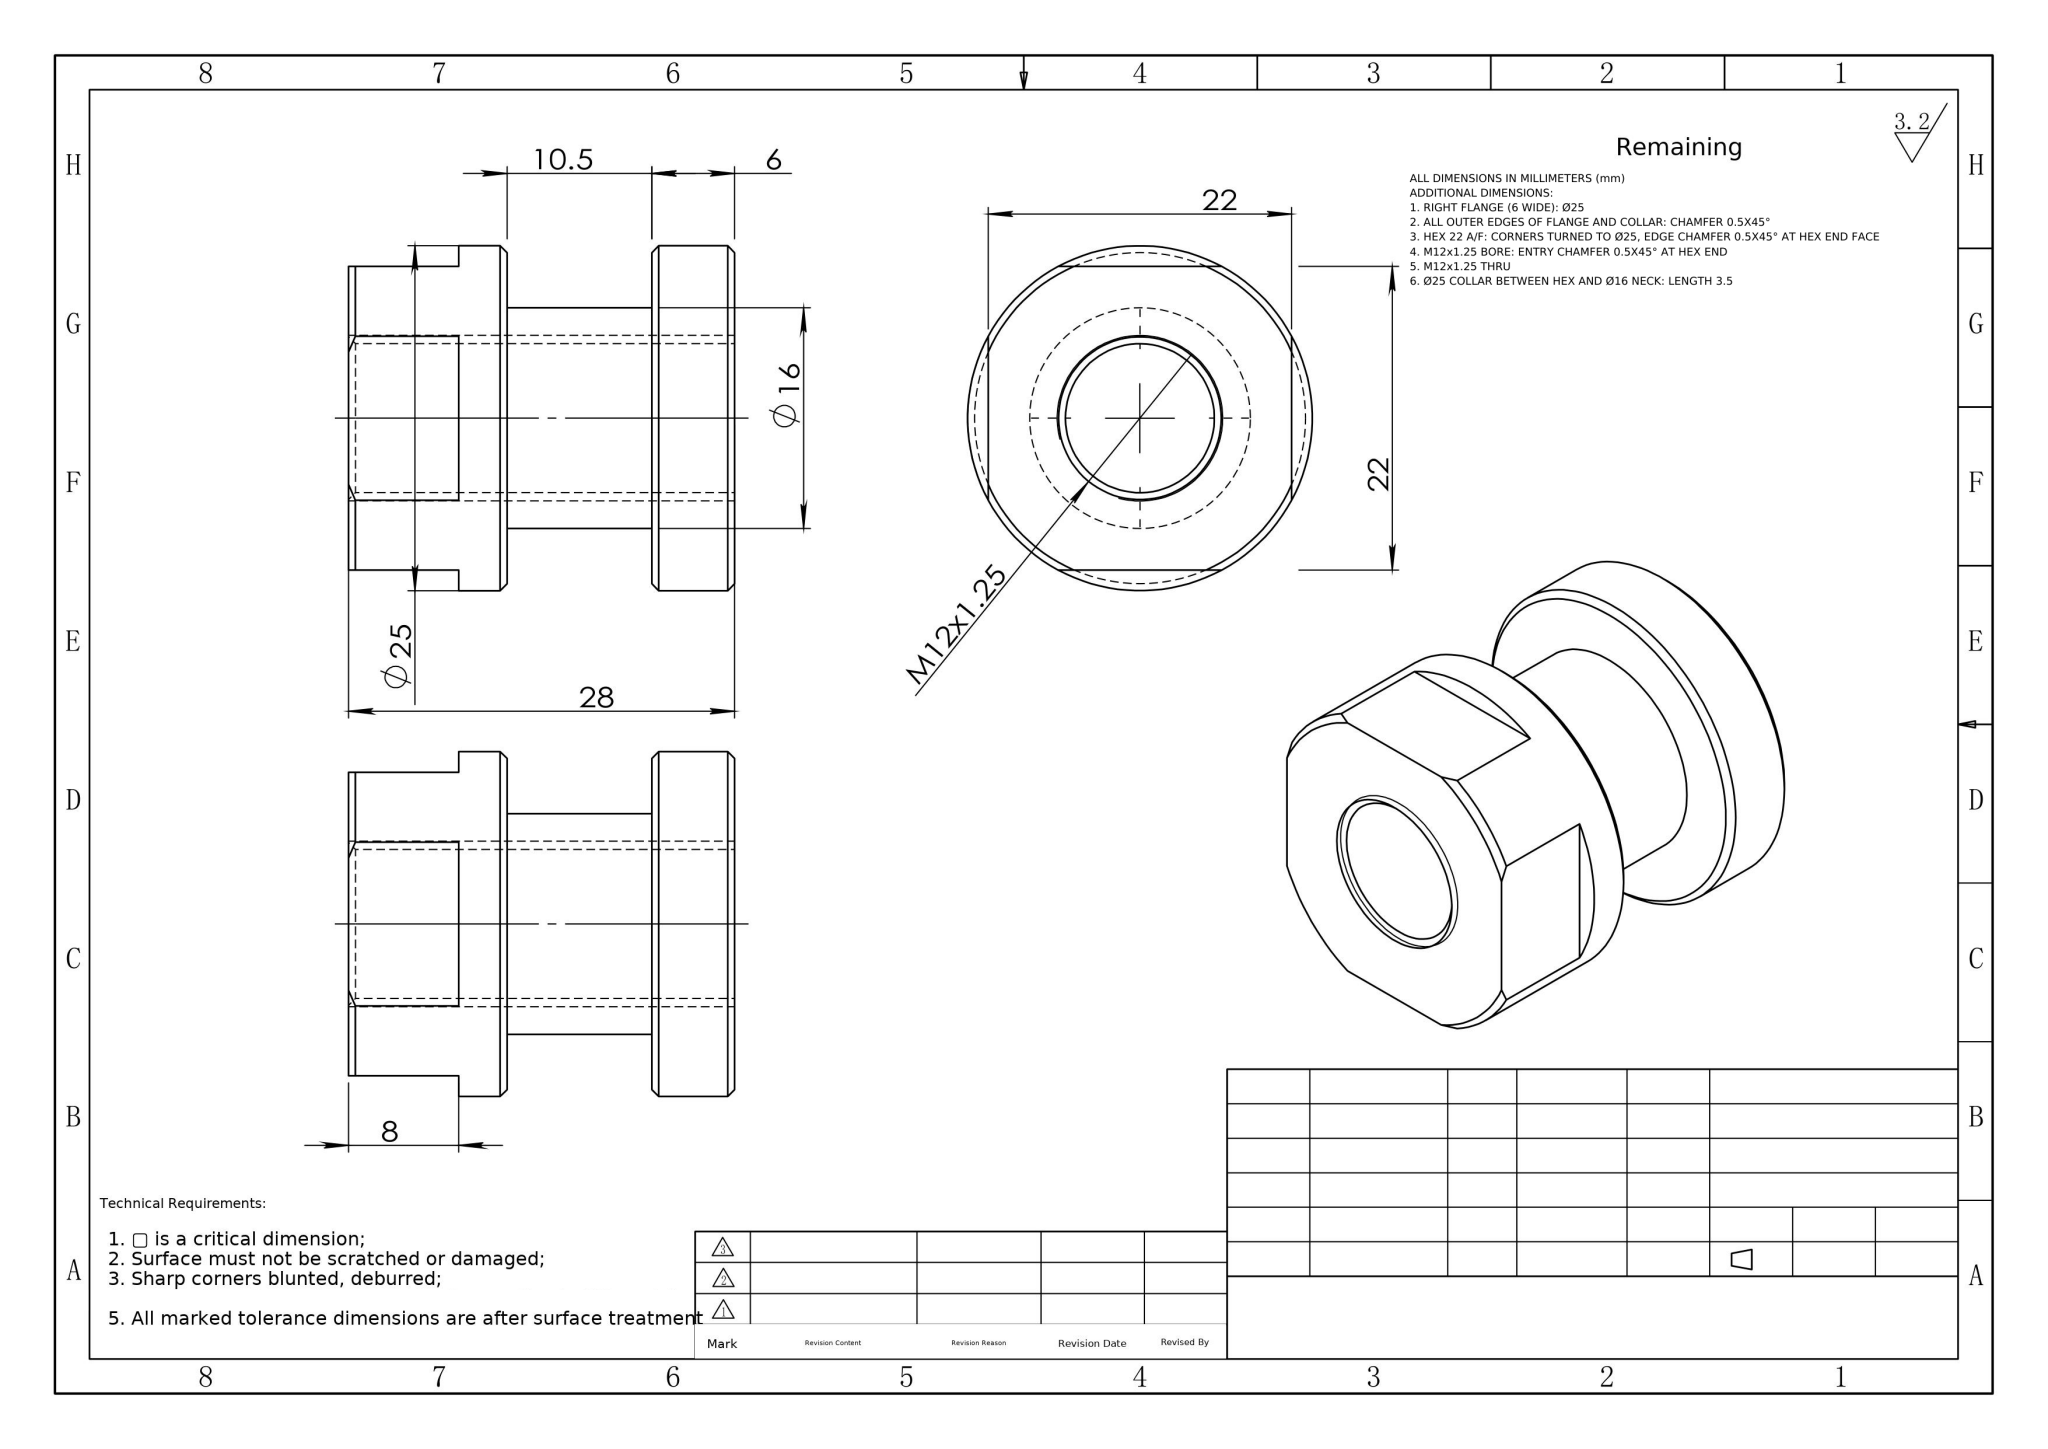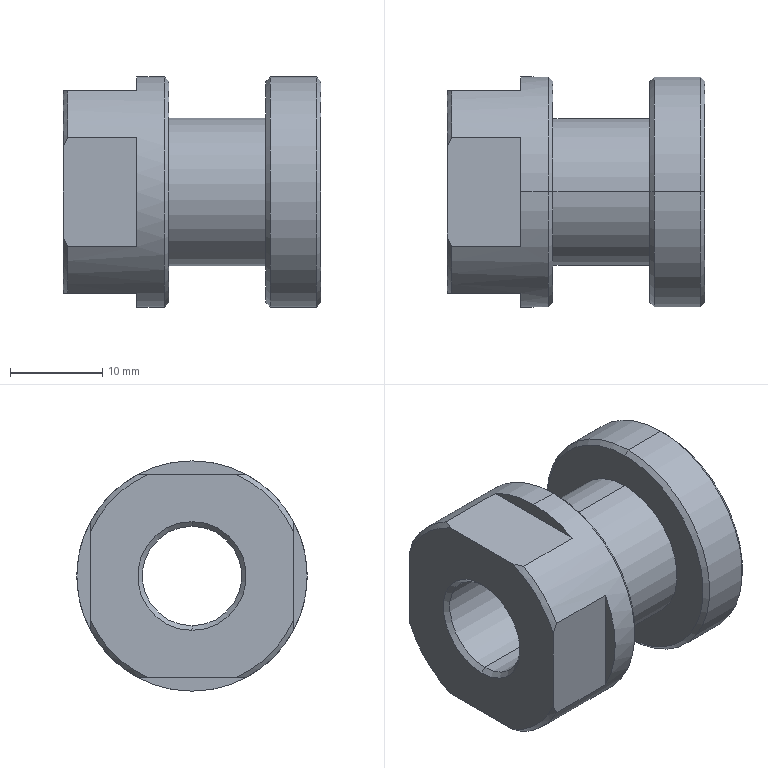Part | NX | mm | 1 solid | 32 faces | box 28 x 25 x 25 mm | volume 7714 mm3 | cone 12 | plane 12 | cylinder 8 | commonest cylinder face diameters 25 x4 10.8 x2 16 x2
STEP:
#1=CARTESIAN_POINT('',(-13.5,0.,-5.4));
#2=VERTEX_POINT('',#1);
#3=CARTESIAN_POINT('',(-13.5,0.,5.4));
#4=VERTEX_POINT('',#3);
#5=CARTESIAN_POINT('',(-13.5,0.,0.));
#6=DIRECTION('',(-1.,0.,0.));
#7=DIRECTION('',(0.,0.,-1.));
#8=AXIS2_PLACEMENT_3D('',#5,#6,#7);
#9=CIRCLE('',#8,5.4);
#10=EDGE_CURVE('',#2,#4,#9,.T.);
#11=ORIENTED_EDGE('',*,*,#10,.F.);
#12=CARTESIAN_POINT('',(-14.,0.,-5.9));
#13=VERTEX_POINT('',#12);
#14=CARTESIAN_POINT('',(-13.5,0.,-5.4));
#15=DIRECTION('',(-0.7071,0.,-0.7071));
#16=VECTOR('',#15,1000.);
#17=LINE('',#14,#16);
#18=EDGE_CURVE('',#2,#13,#17,.T.);
#19=ORIENTED_EDGE('',*,*,#18,.T.);
#20=CARTESIAN_POINT('',(-14.,0.,5.9));
#21=VERTEX_POINT('',#20);
#22=CARTESIAN_POINT('',(-14.,0.,0.));
#23=DIRECTION('',(1.,0.,0.));
#24=DIRECTION('',(0.,0.,-1.));
#25=AXIS2_PLACEMENT_3D('',#22,#23,#24);
#26=CIRCLE('',#25,5.9);
#27=EDGE_CURVE('',#21,#13,#26,.T.);
#28=ORIENTED_EDGE('',*,*,#27,.F.);
#29=CARTESIAN_POINT('',(-13.5,0.,5.4));
#30=DIRECTION('',(-0.7071,0.,0.7071));
#31=VECTOR('',#30,1000.);
#32=LINE('',#29,#31);
#33=EDGE_CURVE('',#4,#21,#32,.T.);
#34=ORIENTED_EDGE('',*,*,#33,.F.);
#35=EDGE_LOOP('',(#11,#19,#28,#34));
#36=FACE_OUTER_BOUND('',#35,.T.);
#37=CARTESIAN_POINT('',(-13.5,0.,0.));
#38=DIRECTION('',(-1.,0.,0.));
#39=DIRECTION('',(0.,0.,1.));
#40=AXIS2_PLACEMENT_3D('',#37,#38,#39);
#41=CONICAL_SURFACE('',#40,5.4,0.7854);
#42=ADVANCED_FACE('',(#36),#41,.F.);
#43=CARTESIAN_POINT('',(8.,0.,12.));
#44=VERTEX_POINT('',#43);
#45=CARTESIAN_POINT('',(8.,0.,-12.));
#46=VERTEX_POINT('',#45);
#47=CARTESIAN_POINT('',(8.,0.,0.));
#48=DIRECTION('',(-1.,0.,0.));
#49=DIRECTION('',(0.,0.,-1.));
#50=AXIS2_PLACEMENT_3D('',#47,#48,#49);
#51=CIRCLE('',#50,12.);
#52=EDGE_CURVE('',#44,#46,#51,.T.);
#53=ORIENTED_EDGE('',*,*,#52,.F.);
#54=CARTESIAN_POINT('',(8.5,0.,12.5));
#55=VERTEX_POINT('',#54);
#56=CARTESIAN_POINT('',(8.,0.,12.));
#57=DIRECTION('',(0.7071,0.,0.7071));
#58=VECTOR('',#57,1000.);
#59=LINE('',#56,#58);
#60=EDGE_CURVE('',#44,#55,#59,.T.);
#61=ORIENTED_EDGE('',*,*,#60,.T.);
#62=CARTESIAN_POINT('',(8.5,0.,-12.5));
#63=VERTEX_POINT('',#62);
#64=CARTESIAN_POINT('',(8.5,0.,0.));
#65=DIRECTION('',(1.,0.,0.));
#66=DIRECTION('',(0.,0.,-1.));
#67=AXIS2_PLACEMENT_3D('',#64,#65,#66);
#68=CIRCLE('',#67,12.5);
#69=EDGE_CURVE('',#63,#55,#68,.T.);
#70=ORIENTED_EDGE('',*,*,#69,.F.);
#71=CARTESIAN_POINT('',(8.,0.,-12.));
#72=DIRECTION('',(0.7071,0.,-0.7071));
#73=VECTOR('',#72,1000.);
#74=LINE('',#71,#73);
#75=EDGE_CURVE('',#46,#63,#74,.T.);
#76=ORIENTED_EDGE('',*,*,#75,.F.);
#77=EDGE_LOOP('',(#53,#61,#70,#76));
#78=FACE_OUTER_BOUND('',#77,.T.);
#79=CARTESIAN_POINT('',(8.,0.,0.));
#80=DIRECTION('',(1.,0.,0.));
#81=DIRECTION('',(0.,0.,-1.));
#82=AXIS2_PLACEMENT_3D('',#79,#80,#81);
#83=CONICAL_SURFACE('',#82,12.,0.7854);
#84=ADVANCED_FACE('',(#78),#83,.T.);
#85=CARTESIAN_POINT('',(-2.5,0.,-12.));
#86=VERTEX_POINT('',#85);
#87=CARTESIAN_POINT('',(-2.5,0.,12.));
#88=VERTEX_POINT('',#87);
#89=CARTESIAN_POINT('',(-2.5,0.,0.));
#90=DIRECTION('',(1.,0.,0.));
#91=DIRECTION('',(0.,0.,1.));
#92=AXIS2_PLACEMENT_3D('',#89,#90,#91);
#93=CIRCLE('',#92,12.);
#94=EDGE_CURVE('',#86,#88,#93,.T.);
#95=ORIENTED_EDGE('',*,*,#94,.F.);
#96=CARTESIAN_POINT('',(-3.,0.,-12.5));
#97=VERTEX_POINT('',#96);
#98=CARTESIAN_POINT('',(-3.,0.,-12.5));
#99=DIRECTION('',(-0.7071,0.,-0.7071));
#100=VECTOR('',#99,1000.);
#101=LINE('',#98,#100);
#102=EDGE_CURVE('',#86,#97,#101,.T.);
#103=ORIENTED_EDGE('',*,*,#102,.T.);
#104=CARTESIAN_POINT('',(-3.,0.,12.5));
#105=VERTEX_POINT('',#104);
#106=CARTESIAN_POINT('',(-3.,0.,0.));
#107=DIRECTION('',(-1.,0.,0.));
#108=DIRECTION('',(0.,0.,1.));
#109=AXIS2_PLACEMENT_3D('',#106,#107,#108);
#110=CIRCLE('',#109,12.5);
#111=EDGE_CURVE('',#105,#97,#110,.T.);
#112=ORIENTED_EDGE('',*,*,#111,.F.);
#113=CARTESIAN_POINT('',(-3.,0.,12.5));
#114=DIRECTION('',(-0.7071,0.,0.7071));
#115=VECTOR('',#114,1000.);
#116=LINE('',#113,#115);
#117=EDGE_CURVE('',#88,#105,#116,.T.);
#118=ORIENTED_EDGE('',*,*,#117,.F.);
#119=EDGE_LOOP('',(#95,#103,#112,#118));
#120=FACE_OUTER_BOUND('',#119,.T.);
#121=CARTESIAN_POINT('',(-3.,0.,0.));
#122=DIRECTION('',(-1.,0.,0.));
#123=DIRECTION('',(0.,0.,1.));
#124=AXIS2_PLACEMENT_3D('',#121,#122,#123);
#125=CONICAL_SURFACE('',#124,12.5,0.7854);
#126=ADVANCED_FACE('',(#120),#125,.T.);
#127=CARTESIAN_POINT('',(14.,0.,-12.));
#128=VERTEX_POINT('',#127);
#129=CARTESIAN_POINT('',(14.,0.,12.));
#130=VERTEX_POINT('',#129);
#131=CARTESIAN_POINT('',(14.,0.,0.));
#132=DIRECTION('',(1.,0.,0.));
#133=DIRECTION('',(0.,0.,1.));
#134=AXIS2_PLACEMENT_3D('',#131,#132,#133);
#135=CIRCLE('',#134,12.);
#136=EDGE_CURVE('',#128,#130,#135,.T.);
#137=ORIENTED_EDGE('',*,*,#136,.F.);
#138=CARTESIAN_POINT('',(13.5,0.,-12.5));
#139=VERTEX_POINT('',#138);
#140=CARTESIAN_POINT('',(13.5,0.,-12.5));
#141=DIRECTION('',(-0.7071,0.,-0.7071));
#142=VECTOR('',#141,1000.);
#143=LINE('',#140,#142);
#144=EDGE_CURVE('',#128,#139,#143,.T.);
#145=ORIENTED_EDGE('',*,*,#144,.T.);
#146=CARTESIAN_POINT('',(13.5,0.,12.5));
#147=VERTEX_POINT('',#146);
#148=CARTESIAN_POINT('',(13.5,0.,0.));
#149=DIRECTION('',(-1.,0.,0.));
#150=DIRECTION('',(0.,0.,1.));
#151=AXIS2_PLACEMENT_3D('',#148,#149,#150);
#152=CIRCLE('',#151,12.5);
#153=EDGE_CURVE('',#147,#139,#152,.T.);
#154=ORIENTED_EDGE('',*,*,#153,.F.);
#155=CARTESIAN_POINT('',(13.5,0.,12.5));
#156=DIRECTION('',(-0.7071,0.,0.7071));
#157=VECTOR('',#156,1000.);
#158=LINE('',#155,#157);
#159=EDGE_CURVE('',#130,#147,#158,.T.);
#160=ORIENTED_EDGE('',*,*,#159,.F.);
#161=EDGE_LOOP('',(#137,#145,#154,#160));
#162=FACE_OUTER_BOUND('',#161,.T.);
#163=CARTESIAN_POINT('',(13.5,0.,0.));
#164=DIRECTION('',(-1.,0.,0.));
#165=DIRECTION('',(0.,0.,1.));
#166=AXIS2_PLACEMENT_3D('',#163,#164,#165);
#167=CONICAL_SURFACE('',#166,12.5,0.7854);
#168=ADVANCED_FACE('',(#162),#167,.T.);
#169=CARTESIAN_POINT('',(14.,0.,-5.4));
#170=VERTEX_POINT('',#169);
#171=CARTESIAN_POINT('',(14.,0.,5.4));
#172=VERTEX_POINT('',#171);
#173=CARTESIAN_POINT('',(14.,0.,0.));
#174=DIRECTION('',(-1.,0.,0.));
#175=DIRECTION('',(0.,0.,1.));
#176=AXIS2_PLACEMENT_3D('',#173,#174,#175);
#177=CIRCLE('',#176,5.4);
#178=EDGE_CURVE('',#170,#172,#177,.T.);
#179=ORIENTED_EDGE('',*,*,#178,.F.);
#180=CARTESIAN_POINT('',(-14.,0.,-5.4));
#181=DIRECTION('',(-1.,0.,0.));
#182=VECTOR('',#181,1000.);
#183=LINE('',#180,#182);
#184=EDGE_CURVE('',#170,#2,#183,.T.);
#185=ORIENTED_EDGE('',*,*,#184,.T.);
#186=ORIENTED_EDGE('',*,*,#10,.T.);
#187=CARTESIAN_POINT('',(-14.,0.,5.4));
#188=DIRECTION('',(-1.,0.,0.));
#189=VECTOR('',#188,1000.);
#190=LINE('',#187,#189);
#191=EDGE_CURVE('',#172,#4,#190,.T.);
#192=ORIENTED_EDGE('',*,*,#191,.F.);
#193=EDGE_LOOP('',(#179,#185,#186,#192));
#194=FACE_OUTER_BOUND('',#193,.T.);
#195=CARTESIAN_POINT('',(-14.,0.,0.));
#196=DIRECTION('',(-1.,0.,0.));
#197=DIRECTION('',(0.,0.,1.));
#198=AXIS2_PLACEMENT_3D('',#195,#196,#197);
#199=CYLINDRICAL_SURFACE('',#198,5.4);
#200=ADVANCED_FACE('',(#194),#199,.F.);
#201=ORIENTED_EDGE('',*,*,#153,.T.);
#202=CARTESIAN_POINT('',(-42.189,0.,-12.5));
#203=DIRECTION('',(-1.,0.,0.));
#204=VECTOR('',#203,1000.);
#205=LINE('',#202,#204);
#206=EDGE_CURVE('',#139,#63,#205,.T.);
#207=ORIENTED_EDGE('',*,*,#206,.T.);
#208=ORIENTED_EDGE('',*,*,#69,.T.);
#209=CARTESIAN_POINT('',(-42.189,0.,12.5));
#210=DIRECTION('',(-1.,0.,0.));
#211=VECTOR('',#210,1000.);
#212=LINE('',#209,#211);
#213=EDGE_CURVE('',#147,#55,#212,.T.);
#214=ORIENTED_EDGE('',*,*,#213,.F.);
#215=EDGE_LOOP('',(#201,#207,#208,#214));
#216=FACE_OUTER_BOUND('',#215,.T.);
#217=CARTESIAN_POINT('',(-42.189,0.,0.));
#218=DIRECTION('',(-1.,0.,0.));
#219=DIRECTION('',(0.,0.,1.));
#220=AXIS2_PLACEMENT_3D('',#217,#218,#219);
#221=CYLINDRICAL_SURFACE('',#220,12.5);
#222=ADVANCED_FACE('',(#216),#221,.T.);
#223=CARTESIAN_POINT('',(8.,0.,8.));
#224=VERTEX_POINT('',#223);
#225=CARTESIAN_POINT('',(8.,0.,-8.));
#226=VERTEX_POINT('',#225);
#227=CARTESIAN_POINT('',(8.,0.,0.));
#228=DIRECTION('',(-1.,0.,0.));
#229=DIRECTION('',(0.,0.,1.));
#230=AXIS2_PLACEMENT_3D('',#227,#228,#229);
#231=CIRCLE('',#230,8.);
#232=EDGE_CURVE('',#224,#226,#231,.T.);
#233=ORIENTED_EDGE('',*,*,#232,.T.);
#234=CARTESIAN_POINT('',(-2.5,0.,-8.));
#235=VERTEX_POINT('',#234);
#236=CARTESIAN_POINT('',(-42.189,0.,-8.));
#237=DIRECTION('',(-1.,0.,0.));
#238=VECTOR('',#237,1000.);
#239=LINE('',#236,#238);
#240=EDGE_CURVE('',#226,#235,#239,.T.);
#241=ORIENTED_EDGE('',*,*,#240,.T.);
#242=CARTESIAN_POINT('',(-2.5,0.,8.));
#243=VERTEX_POINT('',#242);
#244=CARTESIAN_POINT('',(-2.5,0.,0.));
#245=DIRECTION('',(-1.,0.,0.));
#246=DIRECTION('',(0.,0.,1.));
#247=AXIS2_PLACEMENT_3D('',#244,#245,#246);
#248=CIRCLE('',#247,8.);
#249=EDGE_CURVE('',#243,#235,#248,.T.);
#250=ORIENTED_EDGE('',*,*,#249,.F.);
#251=CARTESIAN_POINT('',(-42.189,0.,8.));
#252=DIRECTION('',(-1.,0.,0.));
#253=VECTOR('',#252,1000.);
#254=LINE('',#251,#253);
#255=EDGE_CURVE('',#224,#243,#254,.T.);
#256=ORIENTED_EDGE('',*,*,#255,.F.);
#257=EDGE_LOOP('',(#233,#241,#250,#256));
#258=FACE_OUTER_BOUND('',#257,.T.);
#259=CARTESIAN_POINT('',(-42.189,0.,0.));
#260=DIRECTION('',(-1.,0.,0.));
#261=DIRECTION('',(0.,0.,1.));
#262=AXIS2_PLACEMENT_3D('',#259,#260,#261);
#263=CYLINDRICAL_SURFACE('',#262,8.);
#264=ADVANCED_FACE('',(#258),#263,.T.);
#265=ORIENTED_EDGE('',*,*,#111,.T.);
#266=CARTESIAN_POINT('',(-6.,0.,-12.5));
#267=VERTEX_POINT('',#266);
#268=CARTESIAN_POINT('',(-42.189,0.,-12.5));
#269=DIRECTION('',(-1.,0.,0.));
#270=VECTOR('',#269,1000.);
#271=LINE('',#268,#270);
#272=EDGE_CURVE('',#97,#267,#271,.T.);
#273=ORIENTED_EDGE('',*,*,#272,.T.);
#274=CARTESIAN_POINT('',(-6.,5.937,-11.));
#275=VERTEX_POINT('',#274);
#276=CARTESIAN_POINT('',(-6.,0.,0.));
#277=DIRECTION('',(-1.,0.,0.));
#278=DIRECTION('',(0.,0.,1.));
#279=AXIS2_PLACEMENT_3D('',#276,#277,#278);
#280=CIRCLE('',#279,12.5);
#281=EDGE_CURVE('',#275,#267,#280,.T.);
#282=ORIENTED_EDGE('',*,*,#281,.F.);
#283=CARTESIAN_POINT('',(-13.5,5.937,-11.));
#284=VERTEX_POINT('',#283);
#285=CARTESIAN_POINT('',(-42.189,5.937,-11.));
#286=DIRECTION('',(1.,0.,0.));
#287=VECTOR('',#286,1000.);
#288=LINE('',#285,#287);
#289=EDGE_CURVE('',#284,#275,#288,.T.);
#290=ORIENTED_EDGE('',*,*,#289,.F.);
#291=CARTESIAN_POINT('',(-13.5,11.,-5.937));
#292=VERTEX_POINT('',#291);
#293=CARTESIAN_POINT('',(-13.5,0.,0.));
#294=DIRECTION('',(1.,0.,0.));
#295=DIRECTION('',(0.,0.,-1.));
#296=AXIS2_PLACEMENT_3D('',#293,#294,#295);
#297=CIRCLE('',#296,12.5);
#298=EDGE_CURVE('',#284,#292,#297,.T.);
#299=ORIENTED_EDGE('',*,*,#298,.T.);
#300=CARTESIAN_POINT('',(-6.,11.,-5.937));
#301=VERTEX_POINT('',#300);
#302=CARTESIAN_POINT('',(-42.189,11.,-5.937));
#303=DIRECTION('',(-1.,0.,0.));
#304=VECTOR('',#303,1000.);
#305=LINE('',#302,#304);
#306=EDGE_CURVE('',#301,#292,#305,.T.);
#307=ORIENTED_EDGE('',*,*,#306,.F.);
#308=CARTESIAN_POINT('',(-6.,11.,5.937));
#309=VERTEX_POINT('',#308);
#310=CARTESIAN_POINT('',(-6.,0.,0.));
#311=DIRECTION('',(-1.,0.,0.));
#312=DIRECTION('',(0.,0.,1.));
#313=AXIS2_PLACEMENT_3D('',#310,#311,#312);
#314=CIRCLE('',#313,12.5);
#315=EDGE_CURVE('',#309,#301,#314,.T.);
#316=ORIENTED_EDGE('',*,*,#315,.F.);
#317=CARTESIAN_POINT('',(-13.5,11.,5.937));
#318=VERTEX_POINT('',#317);
#319=CARTESIAN_POINT('',(-42.189,11.,5.937));
#320=DIRECTION('',(1.,0.,0.));
#321=VECTOR('',#320,1000.);
#322=LINE('',#319,#321);
#323=EDGE_CURVE('',#318,#309,#322,.T.);
#324=ORIENTED_EDGE('',*,*,#323,.F.);
#325=CARTESIAN_POINT('',(-13.5,5.937,11.));
#326=VERTEX_POINT('',#325);
#327=CARTESIAN_POINT('',(-13.5,0.,0.));
#328=DIRECTION('',(1.,0.,0.));
#329=DIRECTION('',(0.,0.,-1.));
#330=AXIS2_PLACEMENT_3D('',#327,#328,#329);
#331=CIRCLE('',#330,12.5);
#332=EDGE_CURVE('',#318,#326,#331,.T.);
#333=ORIENTED_EDGE('',*,*,#332,.T.);
#334=CARTESIAN_POINT('',(-6.,5.937,11.));
#335=VERTEX_POINT('',#334);
#336=CARTESIAN_POINT('',(-42.189,5.937,11.));
#337=DIRECTION('',(-1.,0.,0.));
#338=VECTOR('',#337,1000.);
#339=LINE('',#336,#338);
#340=EDGE_CURVE('',#335,#326,#339,.T.);
#341=ORIENTED_EDGE('',*,*,#340,.F.);
#342=CARTESIAN_POINT('',(-6.,0.,12.5));
#343=VERTEX_POINT('',#342);
#344=CARTESIAN_POINT('',(-6.,0.,0.));
#345=DIRECTION('',(-1.,0.,0.));
#346=DIRECTION('',(0.,0.,1.));
#347=AXIS2_PLACEMENT_3D('',#344,#345,#346);
#348=CIRCLE('',#347,12.5);
#349=EDGE_CURVE('',#343,#335,#348,.T.);
#350=ORIENTED_EDGE('',*,*,#349,.F.);
#351=CARTESIAN_POINT('',(-42.189,0.,12.5));
#352=DIRECTION('',(-1.,0.,0.));
#353=VECTOR('',#352,1000.);
#354=LINE('',#351,#353);
#355=EDGE_CURVE('',#105,#343,#354,.T.);
#356=ORIENTED_EDGE('',*,*,#355,.F.);
#357=EDGE_LOOP('',(#265,#273,#282,#290,#299,#307,#316,#324,#333,#341,#350,#356));
#358=FACE_OUTER_BOUND('',#357,.T.);
#359=CARTESIAN_POINT('',(-42.189,0.,0.));
#360=DIRECTION('',(-1.,0.,0.));
#361=DIRECTION('',(0.,0.,1.));
#362=AXIS2_PLACEMENT_3D('',#359,#360,#361);
#363=CYLINDRICAL_SURFACE('',#362,12.5);
#364=ADVANCED_FACE('',(#358),#363,.T.);
#365=ORIENTED_EDGE('',*,*,#27,.T.);
#366=CARTESIAN_POINT('',(-14.,0.,0.));
#367=DIRECTION('',(1.,0.,0.));
#368=DIRECTION('',(0.,0.,-1.));
#369=AXIS2_PLACEMENT_3D('',#366,#367,#368);
#370=CIRCLE('',#369,5.9);
#371=EDGE_CURVE('',#13,#21,#370,.T.);
#372=ORIENTED_EDGE('',*,*,#371,.T.);
#373=EDGE_LOOP('',(#365,#372));
#374=FACE_BOUND('',#373,.T.);
#375=CARTESIAN_POINT('',(-14.,4.796,-11.));
#376=VERTEX_POINT('',#375);
#377=CARTESIAN_POINT('',(-14.,-4.796,-11.));
#378=VERTEX_POINT('',#377);
#379=CARTESIAN_POINT('',(-14.,11.,-11.));
#380=DIRECTION('',(0.,-1.,0.));
#381=VECTOR('',#380,1000.);
#382=LINE('',#379,#381);
#383=EDGE_CURVE('',#376,#378,#382,.T.);
#384=ORIENTED_EDGE('',*,*,#383,.T.);
#385=CARTESIAN_POINT('',(-14.,-11.,-4.796));
#386=VERTEX_POINT('',#385);
#387=CARTESIAN_POINT('',(-14.,0.,0.));
#388=DIRECTION('',(-1.,0.,0.));
#389=DIRECTION('',(0.,0.,-1.));
#390=AXIS2_PLACEMENT_3D('',#387,#388,#389);
#391=CIRCLE('',#390,12.);
#392=EDGE_CURVE('',#378,#386,#391,.T.);
#393=ORIENTED_EDGE('',*,*,#392,.T.);
#394=CARTESIAN_POINT('',(-14.,-11.,4.796));
#395=VERTEX_POINT('',#394);
#396=CARTESIAN_POINT('',(-14.,-11.,-11.));
#397=DIRECTION('',(0.,0.,1.));
#398=VECTOR('',#397,1000.);
#399=LINE('',#396,#398);
#400=EDGE_CURVE('',#386,#395,#399,.T.);
#401=ORIENTED_EDGE('',*,*,#400,.T.);
#402=CARTESIAN_POINT('',(-14.,-4.796,11.));
#403=VERTEX_POINT('',#402);
#404=CARTESIAN_POINT('',(-14.,0.,0.));
#405=DIRECTION('',(-1.,0.,0.));
#406=DIRECTION('',(0.,0.,-1.));
#407=AXIS2_PLACEMENT_3D('',#404,#405,#406);
#408=CIRCLE('',#407,12.);
#409=EDGE_CURVE('',#395,#403,#408,.T.);
#410=ORIENTED_EDGE('',*,*,#409,.T.);
#411=CARTESIAN_POINT('',(-14.,4.796,11.));
#412=VERTEX_POINT('',#411);
#413=CARTESIAN_POINT('',(-14.,11.,11.));
#414=DIRECTION('',(0.,1.,-0.));
#415=VECTOR('',#414,1000.);
#416=LINE('',#413,#415);
#417=EDGE_CURVE('',#403,#412,#416,.T.);
#418=ORIENTED_EDGE('',*,*,#417,.T.);
#419=CARTESIAN_POINT('',(-14.,11.,4.796));
#420=VERTEX_POINT('',#419);
#421=CARTESIAN_POINT('',(-14.,0.,0.));
#422=DIRECTION('',(-1.,0.,0.));
#423=DIRECTION('',(0.,0.,-1.));
#424=AXIS2_PLACEMENT_3D('',#421,#422,#423);
#425=CIRCLE('',#424,12.);
#426=EDGE_CURVE('',#412,#420,#425,.T.);
#427=ORIENTED_EDGE('',*,*,#426,.T.);
#428=CARTESIAN_POINT('',(-14.,11.,-4.796));
#429=VERTEX_POINT('',#428);
#430=CARTESIAN_POINT('',(-14.,11.,-11.));
#431=DIRECTION('',(0.,0.,-1.));
#432=VECTOR('',#431,1000.);
#433=LINE('',#430,#432);
#434=EDGE_CURVE('',#420,#429,#433,.T.);
#435=ORIENTED_EDGE('',*,*,#434,.T.);
#436=CARTESIAN_POINT('',(-14.,0.,0.));
#437=DIRECTION('',(-1.,0.,0.));
#438=DIRECTION('',(0.,0.,-1.));
#439=AXIS2_PLACEMENT_3D('',#436,#437,#438);
#440=CIRCLE('',#439,12.);
#441=EDGE_CURVE('',#429,#376,#440,.T.);
#442=ORIENTED_EDGE('',*,*,#441,.T.);
#443=EDGE_LOOP('',(#384,#393,#401,#410,#418,#427,#435,#442));
#444=FACE_OUTER_BOUND('',#443,.T.);
#445=CARTESIAN_POINT('',(-14.,-0.,0.));
#446=DIRECTION('',(1.,0.,0.));
#447=DIRECTION('',(0.,0.,-1.));
#448=AXIS2_PLACEMENT_3D('',#445,#446,#447);
#449=PLANE('',#448);
#450=ADVANCED_FACE('',(#374,#444),#449,.F.);
#451=ORIENTED_EDGE('',*,*,#272,.F.);
#452=CARTESIAN_POINT('',(-3.,0.,0.));
#453=DIRECTION('',(-1.,0.,0.));
#454=DIRECTION('',(0.,0.,1.));
#455=AXIS2_PLACEMENT_3D('',#452,#453,#454);
#456=CIRCLE('',#455,12.5);
#457=EDGE_CURVE('',#97,#105,#456,.T.);
#458=ORIENTED_EDGE('',*,*,#457,.T.);
#459=ORIENTED_EDGE('',*,*,#355,.T.);
#460=CARTESIAN_POINT('',(-6.,-5.937,11.));
#461=VERTEX_POINT('',#460);
#462=CARTESIAN_POINT('',(-6.,0.,0.));
#463=DIRECTION('',(-1.,0.,0.));
#464=DIRECTION('',(0.,0.,1.));
#465=AXIS2_PLACEMENT_3D('',#462,#463,#464);
#466=CIRCLE('',#465,12.5);
#467=EDGE_CURVE('',#461,#343,#466,.T.);
#468=ORIENTED_EDGE('',*,*,#467,.F.);
#469=CARTESIAN_POINT('',(-13.5,-5.937,11.));
#470=VERTEX_POINT('',#469);
#471=CARTESIAN_POINT('',(-42.189,-5.937,11.));
#472=DIRECTION('',(1.,0.,0.));
#473=VECTOR('',#472,1000.);
#474=LINE('',#471,#473);
#475=EDGE_CURVE('',#470,#461,#474,.T.);
#476=ORIENTED_EDGE('',*,*,#475,.F.);
#477=CARTESIAN_POINT('',(-13.5,-11.,5.937));
#478=VERTEX_POINT('',#477);
#479=CARTESIAN_POINT('',(-13.5,0.,0.));
#480=DIRECTION('',(1.,0.,0.));
#481=DIRECTION('',(0.,0.,-1.));
#482=AXIS2_PLACEMENT_3D('',#479,#480,#481);
#483=CIRCLE('',#482,12.5);
#484=EDGE_CURVE('',#470,#478,#483,.T.);
#485=ORIENTED_EDGE('',*,*,#484,.T.);
#486=CARTESIAN_POINT('',(-6.,-11.,5.937));
#487=VERTEX_POINT('',#486);
#488=CARTESIAN_POINT('',(-42.189,-11.,5.937));
#489=DIRECTION('',(-1.,0.,0.));
#490=VECTOR('',#489,1000.);
#491=LINE('',#488,#490);
#492=EDGE_CURVE('',#487,#478,#491,.T.);
#493=ORIENTED_EDGE('',*,*,#492,.F.);
#494=CARTESIAN_POINT('',(-6.,-11.,-5.937));
#495=VERTEX_POINT('',#494);
#496=CARTESIAN_POINT('',(-6.,0.,0.));
#497=DIRECTION('',(-1.,0.,0.));
#498=DIRECTION('',(0.,0.,1.));
#499=AXIS2_PLACEMENT_3D('',#496,#497,#498);
#500=CIRCLE('',#499,12.5);
#501=EDGE_CURVE('',#495,#487,#500,.T.);
#502=ORIENTED_EDGE('',*,*,#501,.F.);
#503=CARTESIAN_POINT('',(-13.5,-11.,-5.937));
#504=VERTEX_POINT('',#503);
#505=CARTESIAN_POINT('',(-42.189,-11.,-5.937));
#506=DIRECTION('',(1.,0.,0.));
#507=VECTOR('',#506,1000.);
#508=LINE('',#505,#507);
#509=EDGE_CURVE('',#504,#495,#508,.T.);
#510=ORIENTED_EDGE('',*,*,#509,.F.);
#511=CARTESIAN_POINT('',(-13.5,-5.937,-11.));
#512=VERTEX_POINT('',#511);
#513=CARTESIAN_POINT('',(-13.5,0.,0.));
#514=DIRECTION('',(1.,0.,0.));
#515=DIRECTION('',(0.,0.,-1.));
#516=AXIS2_PLACEMENT_3D('',#513,#514,#515);
#517=CIRCLE('',#516,12.5);
#518=EDGE_CURVE('',#504,#512,#517,.T.);
#519=ORIENTED_EDGE('',*,*,#518,.T.);
#520=CARTESIAN_POINT('',(-6.,-5.937,-11.));
#521=VERTEX_POINT('',#520);
#522=CARTESIAN_POINT('',(-42.189,-5.937,-11.));
#523=DIRECTION('',(-1.,0.,0.));
#524=VECTOR('',#523,1000.);
#525=LINE('',#522,#524);
#526=EDGE_CURVE('',#521,#512,#525,.T.);
#527=ORIENTED_EDGE('',*,*,#526,.F.);
#528=CARTESIAN_POINT('',(-6.,0.,0.));
#529=DIRECTION('',(-1.,0.,0.));
#530=DIRECTION('',(0.,0.,1.));
#531=AXIS2_PLACEMENT_3D('',#528,#529,#530);
#532=CIRCLE('',#531,12.5);
#533=EDGE_CURVE('',#267,#521,#532,.T.);
#534=ORIENTED_EDGE('',*,*,#533,.F.);
#535=EDGE_LOOP('',(#451,#458,#459,#468,#476,#485,#493,#502,#510,#519,#527,#534));
#536=FACE_OUTER_BOUND('',#535,.T.);
#537=CARTESIAN_POINT('',(-42.189,0.,0.));
#538=DIRECTION('',(-1.,0.,0.));
#539=DIRECTION('',(0.,0.,1.));
#540=AXIS2_PLACEMENT_3D('',#537,#538,#539);
#541=CYLINDRICAL_SURFACE('',#540,12.5);
#542=ADVANCED_FACE('',(#536),#541,.T.);
#543=CARTESIAN_POINT('',(14.,0.,0.));
#544=DIRECTION('',(1.,0.,0.));
#545=DIRECTION('',(0.,0.,1.));
#546=AXIS2_PLACEMENT_3D('',#543,#544,#545);
#547=CIRCLE('',#546,12.);
#548=EDGE_CURVE('',#130,#128,#547,.T.);
#549=ORIENTED_EDGE('',*,*,#548,.T.);
#550=ORIENTED_EDGE('',*,*,#136,.T.);
#551=EDGE_LOOP('',(#549,#550));
#552=FACE_OUTER_BOUND('',#551,.T.);
#553=CARTESIAN_POINT('',(14.,0.,0.));
#554=DIRECTION('',(-1.,0.,0.));
#555=DIRECTION('',(0.,0.,1.));
#556=AXIS2_PLACEMENT_3D('',#553,#554,#555);
#557=CIRCLE('',#556,5.4);
#558=EDGE_CURVE('',#172,#170,#557,.T.);
#559=ORIENTED_EDGE('',*,*,#558,.T.);
#560=ORIENTED_EDGE('',*,*,#178,.T.);
#561=EDGE_LOOP('',(#559,#560));
#562=FACE_BOUND('',#561,.T.);
#563=CARTESIAN_POINT('',(14.,12.5,0.));
#564=DIRECTION('',(-1.,0.,0.));
#565=DIRECTION('',(0.,0.,1.));
#566=AXIS2_PLACEMENT_3D('',#563,#564,#565);
#567=PLANE('',#566);
#568=ADVANCED_FACE('',(#552,#562),#567,.F.);
#569=CARTESIAN_POINT('',(-2.5,0.,0.));
#570=DIRECTION('',(1.,0.,0.));
#571=DIRECTION('',(0.,0.,1.));
#572=AXIS2_PLACEMENT_3D('',#569,#570,#571);
#573=CIRCLE('',#572,12.);
#574=EDGE_CURVE('',#88,#86,#573,.T.);
#575=ORIENTED_EDGE('',*,*,#574,.T.);
#576=ORIENTED_EDGE('',*,*,#94,.T.);
#577=EDGE_LOOP('',(#575,#576));
#578=FACE_OUTER_BOUND('',#577,.T.);
#579=ORIENTED_EDGE('',*,*,#249,.T.);
#580=CARTESIAN_POINT('',(-2.5,0.,0.));
#581=DIRECTION('',(-1.,0.,0.));
#582=DIRECTION('',(0.,0.,1.));
#583=AXIS2_PLACEMENT_3D('',#580,#581,#582);
#584=CIRCLE('',#583,8.);
#585=EDGE_CURVE('',#235,#243,#584,.T.);
#586=ORIENTED_EDGE('',*,*,#585,.T.);
#587=EDGE_LOOP('',(#579,#586));
#588=FACE_BOUND('',#587,.T.);
#589=CARTESIAN_POINT('',(-2.5,12.5,0.));
#590=DIRECTION('',(-1.,0.,0.));
#591=DIRECTION('',(0.,0.,1.));
#592=AXIS2_PLACEMENT_3D('',#589,#590,#591);
#593=PLANE('',#592);
#594=ADVANCED_FACE('',(#578,#588),#593,.F.);
#595=ORIENTED_EDGE('',*,*,#240,.F.);
#596=CARTESIAN_POINT('',(8.,0.,0.));
#597=DIRECTION('',(-1.,0.,0.));
#598=DIRECTION('',(0.,0.,1.));
#599=AXIS2_PLACEMENT_3D('',#596,#597,#598);
#600=CIRCLE('',#599,8.);
#601=EDGE_CURVE('',#226,#224,#600,.T.);
#602=ORIENTED_EDGE('',*,*,#601,.T.);
#603=ORIENTED_EDGE('',*,*,#255,.T.);
#604=ORIENTED_EDGE('',*,*,#585,.F.);
#605=EDGE_LOOP('',(#595,#602,#603,#604));
#606=FACE_OUTER_BOUND('',#605,.T.);
#607=CARTESIAN_POINT('',(-42.189,0.,0.));
#608=DIRECTION('',(-1.,0.,0.));
#609=DIRECTION('',(0.,0.,1.));
#610=AXIS2_PLACEMENT_3D('',#607,#608,#609);
#611=CYLINDRICAL_SURFACE('',#610,8.);
#612=ADVANCED_FACE('',(#606),#611,.T.);
#613=CARTESIAN_POINT('',(8.,0.,0.));
#614=DIRECTION('',(-1.,0.,0.));
#615=DIRECTION('',(0.,0.,-1.));
#616=AXIS2_PLACEMENT_3D('',#613,#614,#615);
#617=CIRCLE('',#616,12.);
#618=EDGE_CURVE('',#46,#44,#617,.T.);
#619=ORIENTED_EDGE('',*,*,#618,.T.);
#620=ORIENTED_EDGE('',*,*,#52,.T.);
#621=EDGE_LOOP('',(#619,#620));
#622=FACE_OUTER_BOUND('',#621,.T.);
#623=ORIENTED_EDGE('',*,*,#232,.F.);
#624=ORIENTED_EDGE('',*,*,#601,.F.);
#625=EDGE_LOOP('',(#623,#624));
#626=FACE_BOUND('',#625,.T.);
#627=CARTESIAN_POINT('',(8.,12.5,0.));
#628=DIRECTION('',(1.,0.,0.));
#629=DIRECTION('',(0.,0.,-1.));
#630=AXIS2_PLACEMENT_3D('',#627,#628,#629);
#631=PLANE('',#630);
#632=ADVANCED_FACE('',(#622,#626),#631,.F.);
#633=ORIENTED_EDGE('',*,*,#206,.F.);
#634=CARTESIAN_POINT('',(13.5,0.,0.));
#635=DIRECTION('',(-1.,0.,0.));
#636=DIRECTION('',(0.,0.,1.));
#637=AXIS2_PLACEMENT_3D('',#634,#635,#636);
#638=CIRCLE('',#637,12.5);
#639=EDGE_CURVE('',#139,#147,#638,.T.);
#640=ORIENTED_EDGE('',*,*,#639,.T.);
#641=ORIENTED_EDGE('',*,*,#213,.T.);
#642=CARTESIAN_POINT('',(8.5,0.,0.));
#643=DIRECTION('',(1.,0.,0.));
#644=DIRECTION('',(0.,0.,-1.));
#645=AXIS2_PLACEMENT_3D('',#642,#643,#644);
#646=CIRCLE('',#645,12.5);
#647=EDGE_CURVE('',#55,#63,#646,.T.);
#648=ORIENTED_EDGE('',*,*,#647,.T.);
#649=EDGE_LOOP('',(#633,#640,#641,#648));
#650=FACE_OUTER_BOUND('',#649,.T.);
#651=CARTESIAN_POINT('',(-42.189,0.,0.));
#652=DIRECTION('',(-1.,0.,0.));
#653=DIRECTION('',(0.,0.,1.));
#654=AXIS2_PLACEMENT_3D('',#651,#652,#653);
#655=CYLINDRICAL_SURFACE('',#654,12.5);
#656=ADVANCED_FACE('',(#650),#655,.T.);
#657=ORIENTED_EDGE('',*,*,#306,.T.);
#658=CARTESIAN_POINT('',(-13.5,11.,-5.937));
#659=CARTESIAN_POINT('',(-13.678,11.,-5.562));
#660=CARTESIAN_POINT('',(-13.846,11.,-5.182));
#661=CARTESIAN_POINT('',(-14.,11.,-4.796));
#662=B_SPLINE_CURVE_WITH_KNOTS('',3,(#658,#659,#660,#661),.UNSPECIFIED.,.F.,.F.,(4,4),(0.,0.001246),.UNSPECIFIED.);
#663=EDGE_CURVE('',#292,#429,#662,.T.);
#664=ORIENTED_EDGE('',*,*,#663,.T.);
#665=ORIENTED_EDGE('',*,*,#434,.F.);
#666=CARTESIAN_POINT('',(-14.,11.,4.796));
#667=CARTESIAN_POINT('',(-13.846,11.,5.182));
#668=CARTESIAN_POINT('',(-13.678,11.,5.562));
#669=CARTESIAN_POINT('',(-13.5,11.,5.937));
#670=B_SPLINE_CURVE_WITH_KNOTS('',3,(#666,#667,#668,#669),.UNSPECIFIED.,.F.,.F.,(4,4),(0.,0.001246),.UNSPECIFIED.);
#671=EDGE_CURVE('',#420,#318,#670,.T.);
#672=ORIENTED_EDGE('',*,*,#671,.T.);
#673=ORIENTED_EDGE('',*,*,#323,.T.);
#674=CARTESIAN_POINT('',(-6.,11.,-11.));
#675=DIRECTION('',(0.,0.,-1.));
#676=VECTOR('',#675,1000.);
#677=LINE('',#674,#676);
#678=EDGE_CURVE('',#309,#301,#677,.T.);
#679=ORIENTED_EDGE('',*,*,#678,.T.);
#680=EDGE_LOOP('',(#657,#664,#665,#672,#673,#679));
#681=FACE_OUTER_BOUND('',#680,.T.);
#682=CARTESIAN_POINT('',(-6.,11.,-11.));
#683=DIRECTION('',(0.,1.,0.));
#684=DIRECTION('',(0.,0.,1.));
#685=AXIS2_PLACEMENT_3D('',#682,#683,#684);
#686=PLANE('',#685);
#687=ADVANCED_FACE('',(#681),#686,.T.);
#688=ORIENTED_EDGE('',*,*,#315,.T.);
#689=ORIENTED_EDGE('',*,*,#678,.F.);
#690=EDGE_LOOP('',(#688,#689));
#691=FACE_OUTER_BOUND('',#690,.T.);
#692=CARTESIAN_POINT('',(-6.,0.,0.));
#693=DIRECTION('',(-1.,0.,0.));
#694=DIRECTION('',(0.,0.,1.));
#695=AXIS2_PLACEMENT_3D('',#692,#693,#694);
#696=PLANE('',#695);
#697=ADVANCED_FACE('',(#691),#696,.T.);
#698=ORIENTED_EDGE('',*,*,#526,.T.);
#699=CARTESIAN_POINT('',(-13.5,-5.937,-11.));
#700=CARTESIAN_POINT('',(-13.678,-5.562,-11.));
#701=CARTESIAN_POINT('',(-13.846,-5.182,-11.));
#702=CARTESIAN_POINT('',(-14.,-4.796,-11.));
#703=B_SPLINE_CURVE_WITH_KNOTS('',3,(#699,#700,#701,#702),.UNSPECIFIED.,.F.,.F.,(4,4),(0.,0.001246),.UNSPECIFIED.);
#704=EDGE_CURVE('',#512,#378,#703,.T.);
#705=ORIENTED_EDGE('',*,*,#704,.T.);
#706=ORIENTED_EDGE('',*,*,#383,.F.);
#707=CARTESIAN_POINT('',(-14.,4.796,-11.));
#708=CARTESIAN_POINT('',(-13.846,5.182,-11.));
#709=CARTESIAN_POINT('',(-13.678,5.562,-11.));
#710=CARTESIAN_POINT('',(-13.5,5.937,-11.));
#711=B_SPLINE_CURVE_WITH_KNOTS('',3,(#707,#708,#709,#710),.UNSPECIFIED.,.F.,.F.,(4,4),(0.,0.001246),.UNSPECIFIED.);
#712=EDGE_CURVE('',#376,#284,#711,.T.);
#713=ORIENTED_EDGE('',*,*,#712,.T.);
#714=ORIENTED_EDGE('',*,*,#289,.T.);
#715=CARTESIAN_POINT('',(-6.,11.,-11.));
#716=DIRECTION('',(0.,-1.,0.));
#717=VECTOR('',#716,1000.);
#718=LINE('',#715,#717);
#719=EDGE_CURVE('',#275,#521,#718,.T.);
#720=ORIENTED_EDGE('',*,*,#719,.T.);
#721=EDGE_LOOP('',(#698,#705,#706,#713,#714,#720));
#722=FACE_OUTER_BOUND('',#721,.T.);
#723=CARTESIAN_POINT('',(-6.,11.,-11.));
#724=DIRECTION('',(0.,-0.,-1.));
#725=DIRECTION('',(0.,1.,-0.));
#726=AXIS2_PLACEMENT_3D('',#723,#724,#725);
#727=PLANE('',#726);
#728=ADVANCED_FACE('',(#722),#727,.T.);
#729=ORIENTED_EDGE('',*,*,#281,.T.);
#730=ORIENTED_EDGE('',*,*,#533,.T.);
#731=ORIENTED_EDGE('',*,*,#719,.F.);
#732=EDGE_LOOP('',(#729,#730,#731));
#733=FACE_OUTER_BOUND('',#732,.T.);
#734=CARTESIAN_POINT('',(-6.,0.,0.));
#735=DIRECTION('',(-1.,0.,0.));
#736=DIRECTION('',(0.,0.,1.));
#737=AXIS2_PLACEMENT_3D('',#734,#735,#736);
#738=PLANE('',#737);
#739=ADVANCED_FACE('',(#733),#738,.T.);
#740=ORIENTED_EDGE('',*,*,#400,.F.);
#741=CARTESIAN_POINT('',(-14.,-11.,-4.796));
#742=CARTESIAN_POINT('',(-13.846,-11.,-5.182));
#743=CARTESIAN_POINT('',(-13.678,-11.,-5.562));
#744=CARTESIAN_POINT('',(-13.5,-11.,-5.937));
#745=B_SPLINE_CURVE_WITH_KNOTS('',3,(#741,#742,#743,#744),.UNSPECIFIED.,.F.,.F.,(4,4),(0.,0.001246),.UNSPECIFIED.);
#746=EDGE_CURVE('',#386,#504,#745,.T.);
#747=ORIENTED_EDGE('',*,*,#746,.T.);
#748=ORIENTED_EDGE('',*,*,#509,.T.);
#749=CARTESIAN_POINT('',(-6.,-11.,-11.));
#750=DIRECTION('',(0.,0.,1.));
#751=VECTOR('',#750,1000.);
#752=LINE('',#749,#751);
#753=EDGE_CURVE('',#495,#487,#752,.T.);
#754=ORIENTED_EDGE('',*,*,#753,.T.);
#755=ORIENTED_EDGE('',*,*,#492,.T.);
#756=CARTESIAN_POINT('',(-13.5,-11.,5.937));
#757=CARTESIAN_POINT('',(-13.678,-11.,5.562));
#758=CARTESIAN_POINT('',(-13.846,-11.,5.182));
#759=CARTESIAN_POINT('',(-14.,-11.,4.796));
#760=B_SPLINE_CURVE_WITH_KNOTS('',3,(#756,#757,#758,#759),.UNSPECIFIED.,.F.,.F.,(4,4),(0.,0.001246),.UNSPECIFIED.);
#761=EDGE_CURVE('',#478,#395,#760,.T.);
#762=ORIENTED_EDGE('',*,*,#761,.T.);
#763=EDGE_LOOP('',(#740,#747,#748,#754,#755,#762));
#764=FACE_OUTER_BOUND('',#763,.T.);
#765=CARTESIAN_POINT('',(-6.,-11.,-11.));
#766=DIRECTION('',(0.,-1.,0.));
#767=DIRECTION('',(0.,0.,-1.));
#768=AXIS2_PLACEMENT_3D('',#765,#766,#767);
#769=PLANE('',#768);
#770=ADVANCED_FACE('',(#764),#769,.T.);
#771=ORIENTED_EDGE('',*,*,#501,.T.);
#772=ORIENTED_EDGE('',*,*,#753,.F.);
#773=EDGE_LOOP('',(#771,#772));
#774=FACE_OUTER_BOUND('',#773,.T.);
#775=CARTESIAN_POINT('',(-6.,0.,0.));
#776=DIRECTION('',(-1.,0.,0.));
#777=DIRECTION('',(0.,0.,1.));
#778=AXIS2_PLACEMENT_3D('',#775,#776,#777);
#779=PLANE('',#778);
#780=ADVANCED_FACE('',(#774),#779,.T.);
#781=ORIENTED_EDGE('',*,*,#467,.T.);
#782=ORIENTED_EDGE('',*,*,#349,.T.);
#783=CARTESIAN_POINT('',(-6.,11.,11.));
#784=DIRECTION('',(0.,1.,-0.));
#785=VECTOR('',#784,1000.);
#786=LINE('',#783,#785);
#787=EDGE_CURVE('',#461,#335,#786,.T.);
#788=ORIENTED_EDGE('',*,*,#787,.F.);
#789=EDGE_LOOP('',(#781,#782,#788));
#790=FACE_OUTER_BOUND('',#789,.T.);
#791=CARTESIAN_POINT('',(-6.,0.,0.));
#792=DIRECTION('',(-1.,0.,0.));
#793=DIRECTION('',(0.,0.,1.));
#794=AXIS2_PLACEMENT_3D('',#791,#792,#793);
#795=PLANE('',#794);
#796=ADVANCED_FACE('',(#790),#795,.T.);
#797=ORIENTED_EDGE('',*,*,#340,.T.);
#798=CARTESIAN_POINT('',(-13.5,5.937,11.));
#799=CARTESIAN_POINT('',(-13.678,5.562,11.));
#800=CARTESIAN_POINT('',(-13.846,5.182,11.));
#801=CARTESIAN_POINT('',(-14.,4.796,11.));
#802=B_SPLINE_CURVE_WITH_KNOTS('',3,(#798,#799,#800,#801),.UNSPECIFIED.,.F.,.F.,(4,4),(0.,0.001246),.UNSPECIFIED.);
#803=EDGE_CURVE('',#326,#412,#802,.T.);
#804=ORIENTED_EDGE('',*,*,#803,.T.);
#805=ORIENTED_EDGE('',*,*,#417,.F.);
#806=CARTESIAN_POINT('',(-14.,-4.796,11.));
#807=CARTESIAN_POINT('',(-13.846,-5.182,11.));
#808=CARTESIAN_POINT('',(-13.678,-5.562,11.));
#809=CARTESIAN_POINT('',(-13.5,-5.937,11.));
#810=B_SPLINE_CURVE_WITH_KNOTS('',3,(#806,#807,#808,#809),.UNSPECIFIED.,.F.,.F.,(4,4),(0.,0.001246),.UNSPECIFIED.);
#811=EDGE_CURVE('',#403,#470,#810,.T.);
#812=ORIENTED_EDGE('',*,*,#811,.T.);
#813=ORIENTED_EDGE('',*,*,#475,.T.);
#814=ORIENTED_EDGE('',*,*,#787,.T.);
#815=EDGE_LOOP('',(#797,#804,#805,#812,#813,#814));
#816=FACE_OUTER_BOUND('',#815,.T.);
#817=CARTESIAN_POINT('',(-6.,11.,11.));
#818=DIRECTION('',(0.,0.,1.));
#819=DIRECTION('',(0.,-1.,0.));
#820=AXIS2_PLACEMENT_3D('',#817,#818,#819);
#821=PLANE('',#820);
#822=ADVANCED_FACE('',(#816),#821,.T.);
#823=ORIENTED_EDGE('',*,*,#184,.F.);
#824=ORIENTED_EDGE('',*,*,#558,.F.);
#825=ORIENTED_EDGE('',*,*,#191,.T.);
#826=CARTESIAN_POINT('',(-13.5,0.,0.));
#827=DIRECTION('',(-1.,0.,0.));
#828=DIRECTION('',(0.,0.,-1.));
#829=AXIS2_PLACEMENT_3D('',#826,#827,#828);
#830=CIRCLE('',#829,5.4);
#831=EDGE_CURVE('',#4,#2,#830,.T.);
#832=ORIENTED_EDGE('',*,*,#831,.T.);
#833=EDGE_LOOP('',(#823,#824,#825,#832));
#834=FACE_OUTER_BOUND('',#833,.T.);
#835=CARTESIAN_POINT('',(-14.,0.,0.));
#836=DIRECTION('',(-1.,0.,0.));
#837=DIRECTION('',(0.,0.,1.));
#838=AXIS2_PLACEMENT_3D('',#835,#836,#837);
#839=CYLINDRICAL_SURFACE('',#838,5.4);
#840=ADVANCED_FACE('',(#834),#839,.F.);
#841=ORIENTED_EDGE('',*,*,#704,.F.);
#842=ORIENTED_EDGE('',*,*,#518,.F.);
#843=ORIENTED_EDGE('',*,*,#746,.F.);
#844=ORIENTED_EDGE('',*,*,#392,.F.);
#845=EDGE_LOOP('',(#841,#842,#843,#844));
#846=FACE_OUTER_BOUND('',#845,.T.);
#847=CARTESIAN_POINT('',(-14.,0.,0.));
#848=DIRECTION('',(1.,0.,0.));
#849=DIRECTION('',(0.,0.,-1.));
#850=AXIS2_PLACEMENT_3D('',#847,#848,#849);
#851=CONICAL_SURFACE('',#850,12.,0.7854);
#852=ADVANCED_FACE('',(#846),#851,.T.);
#853=ORIENTED_EDGE('',*,*,#663,.F.);
#854=ORIENTED_EDGE('',*,*,#298,.F.);
#855=ORIENTED_EDGE('',*,*,#712,.F.);
#856=ORIENTED_EDGE('',*,*,#441,.F.);
#857=EDGE_LOOP('',(#853,#854,#855,#856));
#858=FACE_OUTER_BOUND('',#857,.T.);
#859=CARTESIAN_POINT('',(-14.,0.,0.));
#860=DIRECTION('',(1.,0.,0.));
#861=DIRECTION('',(0.,0.,-1.));
#862=AXIS2_PLACEMENT_3D('',#859,#860,#861);
#863=CONICAL_SURFACE('',#862,12.,0.7854);
#864=ADVANCED_FACE('',(#858),#863,.T.);
#865=ORIENTED_EDGE('',*,*,#803,.F.);
#866=ORIENTED_EDGE('',*,*,#332,.F.);
#867=ORIENTED_EDGE('',*,*,#671,.F.);
#868=ORIENTED_EDGE('',*,*,#426,.F.);
#869=EDGE_LOOP('',(#865,#866,#867,#868));
#870=FACE_OUTER_BOUND('',#869,.T.);
#871=CARTESIAN_POINT('',(-14.,0.,0.));
#872=DIRECTION('',(1.,0.,0.));
#873=DIRECTION('',(0.,0.,-1.));
#874=AXIS2_PLACEMENT_3D('',#871,#872,#873);
#875=CONICAL_SURFACE('',#874,12.,0.7854);
#876=ADVANCED_FACE('',(#870),#875,.T.);
#877=ORIENTED_EDGE('',*,*,#761,.F.);
#878=ORIENTED_EDGE('',*,*,#484,.F.);
#879=ORIENTED_EDGE('',*,*,#811,.F.);
#880=ORIENTED_EDGE('',*,*,#409,.F.);
#881=EDGE_LOOP('',(#877,#878,#879,#880));
#882=FACE_OUTER_BOUND('',#881,.T.);
#883=CARTESIAN_POINT('',(-14.,0.,0.));
#884=DIRECTION('',(1.,0.,0.));
#885=DIRECTION('',(0.,0.,-1.));
#886=AXIS2_PLACEMENT_3D('',#883,#884,#885);
#887=CONICAL_SURFACE('',#886,12.,0.7854);
#888=ADVANCED_FACE('',(#882),#887,.T.);
#889=ORIENTED_EDGE('',*,*,#144,.F.);
#890=ORIENTED_EDGE('',*,*,#548,.F.);
#891=ORIENTED_EDGE('',*,*,#159,.T.);
#892=ORIENTED_EDGE('',*,*,#639,.F.);
#893=EDGE_LOOP('',(#889,#890,#891,#892));
#894=FACE_OUTER_BOUND('',#893,.T.);
#895=CARTESIAN_POINT('',(13.5,0.,0.));
#896=DIRECTION('',(-1.,0.,0.));
#897=DIRECTION('',(0.,0.,1.));
#898=AXIS2_PLACEMENT_3D('',#895,#896,#897);
#899=CONICAL_SURFACE('',#898,12.5,0.7854);
#900=ADVANCED_FACE('',(#894),#899,.T.);
#901=ORIENTED_EDGE('',*,*,#102,.F.);
#902=ORIENTED_EDGE('',*,*,#574,.F.);
#903=ORIENTED_EDGE('',*,*,#117,.T.);
#904=ORIENTED_EDGE('',*,*,#457,.F.);
#905=EDGE_LOOP('',(#901,#902,#903,#904));
#906=FACE_OUTER_BOUND('',#905,.T.);
#907=CARTESIAN_POINT('',(-3.,0.,0.));
#908=DIRECTION('',(-1.,0.,0.));
#909=DIRECTION('',(0.,0.,1.));
#910=AXIS2_PLACEMENT_3D('',#907,#908,#909);
#911=CONICAL_SURFACE('',#910,12.5,0.7854);
#912=ADVANCED_FACE('',(#906),#911,.T.);
#913=ORIENTED_EDGE('',*,*,#60,.F.);
#914=ORIENTED_EDGE('',*,*,#618,.F.);
#915=ORIENTED_EDGE('',*,*,#75,.T.);
#916=ORIENTED_EDGE('',*,*,#647,.F.);
#917=EDGE_LOOP('',(#913,#914,#915,#916));
#918=FACE_OUTER_BOUND('',#917,.T.);
#919=CARTESIAN_POINT('',(8.,0.,0.));
#920=DIRECTION('',(1.,0.,0.));
#921=DIRECTION('',(0.,0.,-1.));
#922=AXIS2_PLACEMENT_3D('',#919,#920,#921);
#923=CONICAL_SURFACE('',#922,12.,0.7854);
#924=ADVANCED_FACE('',(#918),#923,.T.);
#925=ORIENTED_EDGE('',*,*,#18,.F.);
#926=ORIENTED_EDGE('',*,*,#831,.F.);
#927=ORIENTED_EDGE('',*,*,#33,.T.);
#928=ORIENTED_EDGE('',*,*,#371,.F.);
#929=EDGE_LOOP('',(#925,#926,#927,#928));
#930=FACE_OUTER_BOUND('',#929,.T.);
#931=CARTESIAN_POINT('',(-13.5,0.,0.));
#932=DIRECTION('',(-1.,0.,0.));
#933=DIRECTION('',(0.,0.,1.));
#934=AXIS2_PLACEMENT_3D('',#931,#932,#933);
#935=CONICAL_SURFACE('',#934,5.4,0.7854);
#936=ADVANCED_FACE('',(#930),#935,.F.);
#937=CLOSED_SHELL('',(#42,#84,#126,#168,#200,#222,#264,#364,#450,#542,#568,#594,#612,#632,#656,#687,#697,#728,#739,#770,#780,#796,#822,#840,#852,#864,#876,#888,#900,#912,#924,#936));
#938=MANIFOLD_SOLID_BREP('',#937);
#939=CARTESIAN_POINT('',(0.,0.,0.));
#940=DIRECTION('',(0.,0.,1.));
#941=DIRECTION('',(1.,0.,0.));
#942=AXIS2_PLACEMENT_3D('',#939,#940,#941);
#943=(LENGTH_UNIT()NAMED_UNIT(*)SI_UNIT(.MILLI.,.METRE.));
#944=UNCERTAINTY_MEASURE_WITH_UNIT(LENGTH_MEASURE(0.00001),#943,'','');
#945=(NAMED_UNIT(*)PLANE_ANGLE_UNIT()SI_UNIT($,.RADIAN.));
#946=(NAMED_UNIT(*)SI_UNIT($,.STERADIAN.)SOLID_ANGLE_UNIT());
#947=(GEOMETRIC_REPRESENTATION_CONTEXT(3)GLOBAL_UNCERTAINTY_ASSIGNED_CONTEXT((#944))GLOBAL_UNIT_ASSIGNED_CONTEXT((#943,#945,#946))REPRESENTATION_CONTEXT('',''));
#948=ADVANCED_BREP_SHAPE_REPRESENTATION('',(#938,#942),#947);
#949=COLOUR_RGB('',0.7922,0.8196,0.9333);
#950=FILL_AREA_STYLE_COLOUR('',#949);
#951=FILL_AREA_STYLE('',(#950));
#952=SURFACE_STYLE_FILL_AREA(#951);
#953=SURFACE_SIDE_STYLE('',(#952));
#954=SURFACE_STYLE_USAGE(.BOTH.,#953);
#955=PRESENTATION_STYLE_ASSIGNMENT((#954));
#956=STYLED_ITEM('',(#955),#938);
#957=(LENGTH_UNIT()NAMED_UNIT(*)SI_UNIT(.MILLI.,.METRE.));
#958=UNCERTAINTY_MEASURE_WITH_UNIT(LENGTH_MEASURE(0.00001),#957,'','');
#959=(NAMED_UNIT(*)PLANE_ANGLE_UNIT()SI_UNIT($,.RADIAN.));
#960=(NAMED_UNIT(*)SI_UNIT($,.STERADIAN.)SOLID_ANGLE_UNIT());
#961=(GEOMETRIC_REPRESENTATION_CONTEXT(3)GLOBAL_UNCERTAINTY_ASSIGNED_CONTEXT((#958))GLOBAL_UNIT_ASSIGNED_CONTEXT((#957,#959,#960))REPRESENTATION_CONTEXT('',''));
#962=MECHANICAL_DESIGN_GEOMETRIC_PRESENTATION_REPRESENTATION('',(#956),#961);
#963=PRESENTATION_LAYER_ASSIGNMENT('','',(#956));